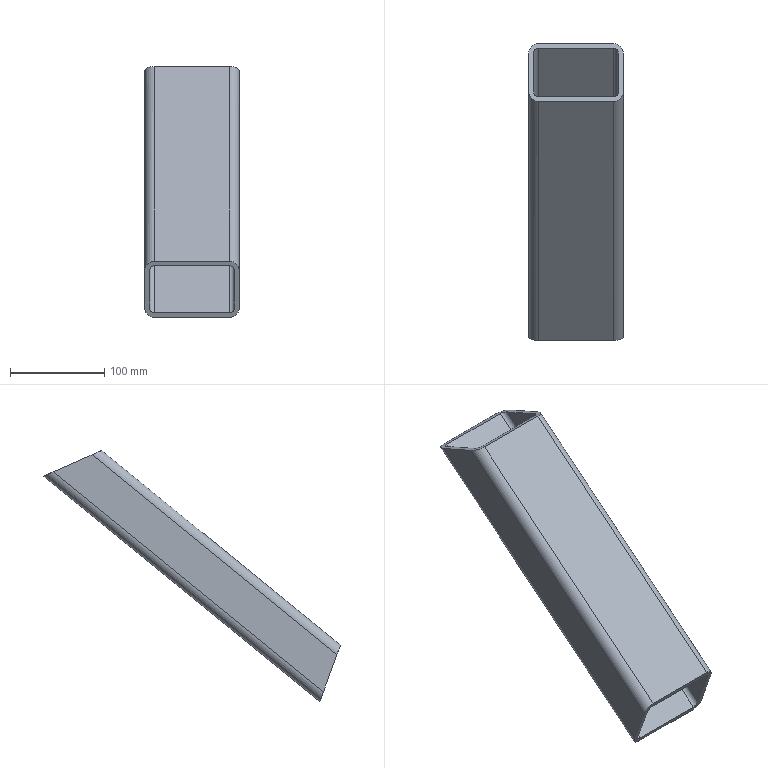Component | SolidWorks | Stap-2-8 | 1 solid | 18 faces | box 100 x 314.75 x 266.08 mm | volume 505822 mm3 | plane 10 | cylinder 8 | commonest cylinder face diameters 20 x4 10 x4 | material Plain Carbon Steel
build123d program:
from build123d import *

# Parameters (mm, degrees)
BOSS_EXTRUDE1_DEPTH = 100
FILLET1_R           = 10
SHELL1_T            = -5


with BuildPart() as part:
    # Sketch1 → Boss-Extrude1 (new body)
    with BuildSketch(Plane.XY):
        Polygon((1451.281, 1386.004), (1382.24, 1757.72), (1328.836, 1716.683), (1388.477, 1395.574), align=None)
    extrude(amount=BOSS_EXTRUDE1_DEPTH)

    # Fillet1
    fillet1_edges = [part.edges().sort_by_distance(p)[0] for p in [
        (1358.657, 1556.128, 100),
        (1358.657, 1556.128, 0),
        (1416.76, 1571.862, 0),
        (1416.76, 1571.862, 100),
    ]]
    fillet(fillet1_edges, radius=FILLET1_R)

    # Shell1
    shell1_openings = [part.faces().sort_by_distance(p)[0] for p in [
        (1355.538, 1737.202, 50),
        (1419.879, 1390.789, 50),
    ]]
    offset(amount=SHELL1_T, openings=shell1_openings, kind=Kind.INTERSECTION)


solid = part.part

# Placed as in the assembly
solid = solid.moved(Location((-124, -2903.176, 779.332), (28.67, 90, 0)))
STEP:
#1=COLOUR_RGB('',0.7922,0.8196,0.9333);
#2=FILL_AREA_STYLE_COLOUR('',#1);
#3=FILL_AREA_STYLE('',(#2));
#4=SURFACE_STYLE_FILL_AREA(#3);
#5=SURFACE_SIDE_STYLE('',(#4));
#6=SURFACE_STYLE_USAGE(.BOTH.,#5);
#7=PRESENTATION_STYLE_ASSIGNMENT((#6));
#8=CARTESIAN_POINT('',(-4.685,-39.722,8.689));
#9=VERTEX_POINT('',#8);
#10=CARTESIAN_POINT('',(-4.685,-39.151,7.122));
#11=VERTEX_POINT('',#10);
#12=CARTESIAN_POINT('',(-4.685,-39.865,9.08));
#13=DIRECTION('',(0.,0.3421,-0.9397));
#14=VECTOR('',#13,39.37);
#15=LINE('',#12,#14);
#16=EDGE_CURVE('',#9,#11,#15,.T.);
#17=ORIENTED_EDGE('',*,*,#16,.F.);
#18=CARTESIAN_POINT('',(-4.488,-39.793,8.884));
#19=VERTEX_POINT('',#18);
#20=CARTESIAN_POINT('',(-4.488,-39.793,8.884));
#21=CARTESIAN_POINT('',(-4.604,-39.793,8.884));
#22=CARTESIAN_POINT('',(-4.685,-39.764,8.803));
#23=CARTESIAN_POINT('',(-4.685,-39.722,8.689));
#24=(BOUNDED_CURVE()B_SPLINE_CURVE(3,(#20,#21,#22,#23),.UNSPECIFIED.,.F.,.T.)B_SPLINE_CURVE_WITH_KNOTS((4,4),(3.142,4.712),.UNSPECIFIED.)CURVE()GEOMETRIC_REPRESENTATION_ITEM()RATIONAL_B_SPLINE_CURVE((1.,0.8047,0.8047,1.))REPRESENTATION_ITEM(''));
#25=EDGE_CURVE('',#19,#9,#24,.T.);
#26=ORIENTED_EDGE('',*,*,#25,.F.);
#27=CARTESIAN_POINT('',(-1.339,-39.793,8.884));
#28=VERTEX_POINT('',#27);
#29=CARTESIAN_POINT('',(-0.9449,-39.793,8.884));
#30=DIRECTION('',(-1.,0.,-0.));
#31=VECTOR('',#30,39.37);
#32=LINE('',#29,#31);
#33=EDGE_CURVE('',#28,#19,#32,.T.);
#34=ORIENTED_EDGE('',*,*,#33,.F.);
#35=CARTESIAN_POINT('',(-1.142,-39.722,8.689));
#36=VERTEX_POINT('',#35);
#37=CARTESIAN_POINT('',(-1.142,-39.722,8.689));
#38=CARTESIAN_POINT('',(-1.142,-39.764,8.803));
#39=CARTESIAN_POINT('',(-1.223,-39.793,8.884));
#40=CARTESIAN_POINT('',(-1.339,-39.793,8.884));
#41=(BOUNDED_CURVE()B_SPLINE_CURVE(3,(#37,#38,#39,#40),.UNSPECIFIED.,.F.,.F.)B_SPLINE_CURVE_WITH_KNOTS((4,4),(4.712,6.283),.UNSPECIFIED.)CURVE()GEOMETRIC_REPRESENTATION_ITEM()RATIONAL_B_SPLINE_CURVE((1.,0.8047,0.8047,1.))REPRESENTATION_ITEM(''));
#42=EDGE_CURVE('',#36,#28,#41,.T.);
#43=ORIENTED_EDGE('',*,*,#42,.F.);
#44=CARTESIAN_POINT('',(-1.142,-39.151,7.122));
#45=VERTEX_POINT('',#44);
#46=CARTESIAN_POINT('',(-1.142,-39.865,9.08));
#47=DIRECTION('',(0.,0.3421,-0.9397));
#48=VECTOR('',#47,39.37);
#49=LINE('',#46,#48);
#50=EDGE_CURVE('',#36,#45,#49,.T.);
#51=ORIENTED_EDGE('',*,*,#50,.T.);
#52=CARTESIAN_POINT('',(-1.339,-39.08,6.926));
#53=VERTEX_POINT('',#52);
#54=CARTESIAN_POINT('',(-1.339,-39.08,6.926));
#55=CARTESIAN_POINT('',(-1.223,-39.08,6.926));
#56=CARTESIAN_POINT('',(-1.142,-39.11,7.007));
#57=CARTESIAN_POINT('',(-1.142,-39.151,7.122));
#58=(BOUNDED_CURVE()B_SPLINE_CURVE(3,(#54,#55,#56,#57),.UNSPECIFIED.,.F.,.F.)B_SPLINE_CURVE_WITH_KNOTS((4,4),(0.,1.571),.UNSPECIFIED.)CURVE()GEOMETRIC_REPRESENTATION_ITEM()RATIONAL_B_SPLINE_CURVE((1.,0.8047,0.8047,1.))REPRESENTATION_ITEM(''));
#59=EDGE_CURVE('',#53,#45,#58,.T.);
#60=ORIENTED_EDGE('',*,*,#59,.F.);
#61=CARTESIAN_POINT('',(-4.488,-39.08,6.926));
#62=VERTEX_POINT('',#61);
#63=CARTESIAN_POINT('',(-0.9449,-39.08,6.926));
#64=DIRECTION('',(-1.,0.,-0.));
#65=VECTOR('',#64,39.37);
#66=LINE('',#63,#65);
#67=EDGE_CURVE('',#53,#62,#66,.T.);
#68=ORIENTED_EDGE('',*,*,#67,.T.);
#69=CARTESIAN_POINT('',(-4.685,-39.151,7.122));
#70=CARTESIAN_POINT('',(-4.685,-39.11,7.007));
#71=CARTESIAN_POINT('',(-4.604,-39.08,6.926));
#72=CARTESIAN_POINT('',(-4.488,-39.08,6.926));
#73=(BOUNDED_CURVE()B_SPLINE_CURVE(3,(#69,#70,#71,#72),.UNSPECIFIED.,.F.,.T.)B_SPLINE_CURVE_WITH_KNOTS((4,4),(1.571,3.142),.UNSPECIFIED.)CURVE()GEOMETRIC_REPRESENTATION_ITEM()RATIONAL_B_SPLINE_CURVE((1.,0.8047,0.8047,1.))REPRESENTATION_ITEM(''));
#74=EDGE_CURVE('',#11,#62,#73,.T.);
#75=ORIENTED_EDGE('',*,*,#74,.F.);
#76=EDGE_LOOP('',(#17,#26,#34,#43,#51,#60,#68,#75));
#77=FACE_BOUND('',#76,.T.);
#78=CARTESIAN_POINT('',(-4.882,-39.722,8.689));
#79=VERTEX_POINT('',#78);
#80=CARTESIAN_POINT('',(-4.882,-39.151,7.122));
#81=VERTEX_POINT('',#80);
#82=CARTESIAN_POINT('',(-4.882,-39.865,9.08));
#83=DIRECTION('',(0.,0.3421,-0.9397));
#84=VECTOR('',#83,39.37);
#85=LINE('',#82,#84);
#86=EDGE_CURVE('',#79,#81,#85,.T.);
#87=ORIENTED_EDGE('',*,*,#86,.T.);
#88=CARTESIAN_POINT('',(-4.488,-39.009,6.73));
#89=VERTEX_POINT('',#88);
#90=CARTESIAN_POINT('',(-4.882,-39.151,7.122));
#91=CARTESIAN_POINT('',(-4.882,-39.068,6.892));
#92=CARTESIAN_POINT('',(-4.719,-39.009,6.73));
#93=CARTESIAN_POINT('',(-4.488,-39.009,6.73));
#94=(BOUNDED_CURVE()B_SPLINE_CURVE(3,(#90,#91,#92,#93),.UNSPECIFIED.,.F.,.T.)B_SPLINE_CURVE_WITH_KNOTS((4,4),(1.571,3.142),.UNSPECIFIED.)CURVE()GEOMETRIC_REPRESENTATION_ITEM()RATIONAL_B_SPLINE_CURVE((1.,0.8047,0.8047,1.))REPRESENTATION_ITEM(''));
#95=EDGE_CURVE('',#81,#89,#94,.T.);
#96=ORIENTED_EDGE('',*,*,#95,.T.);
#97=CARTESIAN_POINT('',(-1.339,-39.009,6.73));
#98=VERTEX_POINT('',#97);
#99=CARTESIAN_POINT('',(-0.9449,-39.009,6.73));
#100=DIRECTION('',(-1.,0.,-0.));
#101=VECTOR('',#100,39.37);
#102=LINE('',#99,#101);
#103=EDGE_CURVE('',#98,#89,#102,.T.);
#104=ORIENTED_EDGE('',*,*,#103,.F.);
#105=CARTESIAN_POINT('',(-0.9449,-39.151,7.122));
#106=VERTEX_POINT('',#105);
#107=CARTESIAN_POINT('',(-1.339,-39.009,6.73));
#108=CARTESIAN_POINT('',(-1.108,-39.009,6.73));
#109=CARTESIAN_POINT('',(-0.9449,-39.068,6.892));
#110=CARTESIAN_POINT('',(-0.9449,-39.151,7.122));
#111=(BOUNDED_CURVE()B_SPLINE_CURVE(3,(#107,#108,#109,#110),.UNSPECIFIED.,.F.,.F.)B_SPLINE_CURVE_WITH_KNOTS((4,4),(0.,1.571),.UNSPECIFIED.)CURVE()GEOMETRIC_REPRESENTATION_ITEM()RATIONAL_B_SPLINE_CURVE((1.,0.8047,0.8047,1.))REPRESENTATION_ITEM(''));
#112=EDGE_CURVE('',#98,#106,#111,.T.);
#113=ORIENTED_EDGE('',*,*,#112,.T.);
#114=CARTESIAN_POINT('',(-0.9449,-39.722,8.689));
#115=VERTEX_POINT('',#114);
#116=CARTESIAN_POINT('',(-0.9449,-39.865,9.08));
#117=DIRECTION('',(0.,0.3421,-0.9397));
#118=VECTOR('',#117,39.37);
#119=LINE('',#116,#118);
#120=EDGE_CURVE('',#115,#106,#119,.T.);
#121=ORIENTED_EDGE('',*,*,#120,.F.);
#122=CARTESIAN_POINT('',(-1.339,-39.865,9.08));
#123=VERTEX_POINT('',#122);
#124=CARTESIAN_POINT('',(-0.9449,-39.722,8.689));
#125=CARTESIAN_POINT('',(-0.9449,-39.805,8.918));
#126=CARTESIAN_POINT('',(-1.108,-39.865,9.08));
#127=CARTESIAN_POINT('',(-1.339,-39.865,9.08));
#128=(BOUNDED_CURVE()B_SPLINE_CURVE(3,(#124,#125,#126,#127),.UNSPECIFIED.,.F.,.T.)B_SPLINE_CURVE_WITH_KNOTS((4,4),(4.712,6.283),.UNSPECIFIED.)CURVE()GEOMETRIC_REPRESENTATION_ITEM()RATIONAL_B_SPLINE_CURVE((1.,0.8047,0.8047,1.))REPRESENTATION_ITEM(''));
#129=EDGE_CURVE('',#115,#123,#128,.T.);
#130=ORIENTED_EDGE('',*,*,#129,.T.);
#131=CARTESIAN_POINT('',(-4.488,-39.865,9.08));
#132=VERTEX_POINT('',#131);
#133=CARTESIAN_POINT('',(-0.9449,-39.865,9.08));
#134=DIRECTION('',(-1.,0.,-0.));
#135=VECTOR('',#134,39.37);
#136=LINE('',#133,#135);
#137=EDGE_CURVE('',#123,#132,#136,.T.);
#138=ORIENTED_EDGE('',*,*,#137,.T.);
#139=CARTESIAN_POINT('',(-4.488,-39.865,9.08));
#140=CARTESIAN_POINT('',(-4.719,-39.865,9.08));
#141=CARTESIAN_POINT('',(-4.882,-39.805,8.918));
#142=CARTESIAN_POINT('',(-4.882,-39.722,8.689));
#143=(BOUNDED_CURVE()B_SPLINE_CURVE(3,(#139,#140,#141,#142),.UNSPECIFIED.,.F.,.F.)B_SPLINE_CURVE_WITH_KNOTS((4,4),(3.142,4.712),.UNSPECIFIED.)CURVE()GEOMETRIC_REPRESENTATION_ITEM()RATIONAL_B_SPLINE_CURVE((1.,0.8047,0.8047,1.))REPRESENTATION_ITEM(''));
#144=EDGE_CURVE('',#132,#79,#143,.T.);
#145=ORIENTED_EDGE('',*,*,#144,.T.);
#146=EDGE_LOOP('',(#87,#96,#104,#113,#121,#130,#138,#145));
#147=FACE_OUTER_BOUND('',#146,.T.);
#148=CARTESIAN_POINT('',(-0.9449,-39.865,9.08));
#149=DIRECTION('',(-0.,0.9397,0.3421));
#150=DIRECTION('',(-0.,-0.3421,0.9397));
#151=AXIS2_PLACEMENT_3D('',#148,#149,#150);
#152=PLANE('',#151);
#153=ADVANCED_FACE('',(#77,#147),#152,.F.);
#154=ORIENTED_EDGE('',*,*,#103,.T.);
#155=CARTESIAN_POINT('',(-4.488,-27.473,16.136));
#156=VERTEX_POINT('',#155);
#157=CARTESIAN_POINT('',(-4.488,-39.009,6.73));
#158=DIRECTION('',(-0.,0.775,0.6319));
#159=VECTOR('',#158,39.37);
#160=LINE('',#157,#159);
#161=EDGE_CURVE('',#89,#156,#160,.T.);
#162=ORIENTED_EDGE('',*,*,#161,.T.);
#163=CARTESIAN_POINT('',(-1.339,-27.473,16.136));
#164=VERTEX_POINT('',#163);
#165=CARTESIAN_POINT('',(-0.9449,-27.473,16.136));
#166=DIRECTION('',(-1.,0.,-0.));
#167=VECTOR('',#166,39.37);
#168=LINE('',#165,#167);
#169=EDGE_CURVE('',#164,#156,#168,.T.);
#170=ORIENTED_EDGE('',*,*,#169,.F.);
#171=CARTESIAN_POINT('',(-1.339,-39.009,6.73));
#172=DIRECTION('',(0.,-0.775,-0.6319));
#173=VECTOR('',#172,39.37);
#174=LINE('',#171,#173);
#175=EDGE_CURVE('',#164,#98,#174,.T.);
#176=ORIENTED_EDGE('',*,*,#175,.T.);
#177=EDGE_LOOP('',(#154,#162,#170,#176));
#178=FACE_OUTER_BOUND('',#177,.T.);
#179=CARTESIAN_POINT('',(-0.9449,-39.009,6.73));
#180=DIRECTION('',(-0.,-0.6319,0.775));
#181=DIRECTION('',(0.,-0.775,-0.6319));
#182=AXIS2_PLACEMENT_3D('',#179,#180,#181);
#183=PLANE('',#182);
#184=ADVANCED_FACE('',(#178),#183,.F.);
#185=CARTESIAN_POINT('',(-1.339,-27.675,16.225));
#186=VERTEX_POINT('',#185);
#187=CARTESIAN_POINT('',(-4.488,-27.675,16.225));
#188=VERTEX_POINT('',#187);
#189=CARTESIAN_POINT('',(-0.9449,-27.675,16.225));
#190=DIRECTION('',(-1.,0.,-0.));
#191=VECTOR('',#190,39.37);
#192=LINE('',#189,#191);
#193=EDGE_CURVE('',#186,#188,#192,.T.);
#194=ORIENTED_EDGE('',*,*,#193,.F.);
#195=CARTESIAN_POINT('',(-1.142,-27.877,16.314));
#196=VERTEX_POINT('',#195);
#197=CARTESIAN_POINT('',(-1.142,-27.877,16.314));
#198=CARTESIAN_POINT('',(-1.142,-27.759,16.262));
#199=CARTESIAN_POINT('',(-1.223,-27.675,16.225));
#200=CARTESIAN_POINT('',(-1.339,-27.675,16.225));
#201=(BOUNDED_CURVE()B_SPLINE_CURVE(3,(#197,#198,#199,#200),.UNSPECIFIED.,.F.,.T.)B_SPLINE_CURVE_WITH_KNOTS((4,4),(1.571,3.142),.UNSPECIFIED.)CURVE()GEOMETRIC_REPRESENTATION_ITEM()RATIONAL_B_SPLINE_CURVE((1.,0.8047,0.8047,1.))REPRESENTATION_ITEM(''));
#202=EDGE_CURVE('',#196,#186,#201,.T.);
#203=ORIENTED_EDGE('',*,*,#202,.F.);
#204=CARTESIAN_POINT('',(-1.142,-29.495,17.027));
#205=VERTEX_POINT('',#204);
#206=CARTESIAN_POINT('',(-1.142,-27.473,16.136));
#207=DIRECTION('',(-0.,-0.915,0.4034));
#208=VECTOR('',#207,39.37);
#209=LINE('',#206,#208);
#210=EDGE_CURVE('',#196,#205,#209,.T.);
#211=ORIENTED_EDGE('',*,*,#210,.T.);
#212=CARTESIAN_POINT('',(-1.339,-29.697,17.117));
#213=VERTEX_POINT('',#212);
#214=CARTESIAN_POINT('',(-1.339,-29.697,17.117));
#215=CARTESIAN_POINT('',(-1.223,-29.697,17.117));
#216=CARTESIAN_POINT('',(-1.142,-29.613,17.08));
#217=CARTESIAN_POINT('',(-1.142,-29.495,17.027));
#218=(BOUNDED_CURVE()B_SPLINE_CURVE(3,(#214,#215,#216,#217),.UNSPECIFIED.,.F.,.T.)B_SPLINE_CURVE_WITH_KNOTS((4,4),(3.142,4.712),.UNSPECIFIED.)CURVE()GEOMETRIC_REPRESENTATION_ITEM()RATIONAL_B_SPLINE_CURVE((1.,0.8047,0.8047,1.))REPRESENTATION_ITEM(''));
#219=EDGE_CURVE('',#213,#205,#218,.T.);
#220=ORIENTED_EDGE('',*,*,#219,.F.);
#221=CARTESIAN_POINT('',(-4.488,-29.697,17.117));
#222=VERTEX_POINT('',#221);
#223=CARTESIAN_POINT('',(-0.9449,-29.697,17.117));
#224=DIRECTION('',(-1.,0.,-0.));
#225=VECTOR('',#224,39.37);
#226=LINE('',#223,#225);
#227=EDGE_CURVE('',#213,#222,#226,.T.);
#228=ORIENTED_EDGE('',*,*,#227,.T.);
#229=CARTESIAN_POINT('',(-4.685,-29.495,17.027));
#230=VERTEX_POINT('',#229);
#231=CARTESIAN_POINT('',(-4.685,-29.495,17.027));
#232=CARTESIAN_POINT('',(-4.685,-29.613,17.08));
#233=CARTESIAN_POINT('',(-4.604,-29.697,17.117));
#234=CARTESIAN_POINT('',(-4.488,-29.697,17.117));
#235=(BOUNDED_CURVE()B_SPLINE_CURVE(3,(#231,#232,#233,#234),.UNSPECIFIED.,.F.,.T.)B_SPLINE_CURVE_WITH_KNOTS((4,4),(4.712,6.283),.UNSPECIFIED.)CURVE()GEOMETRIC_REPRESENTATION_ITEM()RATIONAL_B_SPLINE_CURVE((1.,0.8047,0.8047,1.))REPRESENTATION_ITEM(''));
#236=EDGE_CURVE('',#230,#222,#235,.T.);
#237=ORIENTED_EDGE('',*,*,#236,.F.);
#238=CARTESIAN_POINT('',(-4.685,-27.877,16.314));
#239=VERTEX_POINT('',#238);
#240=CARTESIAN_POINT('',(-4.685,-27.473,16.136));
#241=DIRECTION('',(-0.,-0.915,0.4034));
#242=VECTOR('',#241,39.37);
#243=LINE('',#240,#242);
#244=EDGE_CURVE('',#239,#230,#243,.T.);
#245=ORIENTED_EDGE('',*,*,#244,.F.);
#246=CARTESIAN_POINT('',(-4.488,-27.675,16.225));
#247=CARTESIAN_POINT('',(-4.604,-27.675,16.225));
#248=CARTESIAN_POINT('',(-4.685,-27.759,16.262));
#249=CARTESIAN_POINT('',(-4.685,-27.877,16.314));
#250=(BOUNDED_CURVE()B_SPLINE_CURVE(3,(#246,#247,#248,#249),.UNSPECIFIED.,.F.,.T.)B_SPLINE_CURVE_WITH_KNOTS((4,4),(0.,1.571),.UNSPECIFIED.)CURVE()GEOMETRIC_REPRESENTATION_ITEM()RATIONAL_B_SPLINE_CURVE((1.,0.8047,0.8047,1.))REPRESENTATION_ITEM(''));
#251=EDGE_CURVE('',#188,#239,#250,.T.);
#252=ORIENTED_EDGE('',*,*,#251,.F.);
#253=EDGE_LOOP('',(#194,#203,#211,#220,#228,#237,#245,#252));
#254=FACE_BOUND('',#253,.T.);
#255=ORIENTED_EDGE('',*,*,#169,.T.);
#256=CARTESIAN_POINT('',(-4.882,-27.877,16.314));
#257=VERTEX_POINT('',#256);
#258=CARTESIAN_POINT('',(-4.488,-27.473,16.136));
#259=CARTESIAN_POINT('',(-4.719,-27.473,16.136));
#260=CARTESIAN_POINT('',(-4.882,-27.64,16.21));
#261=CARTESIAN_POINT('',(-4.882,-27.877,16.314));
#262=(BOUNDED_CURVE()B_SPLINE_CURVE(3,(#258,#259,#260,#261),.UNSPECIFIED.,.F.,.F.)B_SPLINE_CURVE_WITH_KNOTS((4,4),(0.,1.571),.UNSPECIFIED.)CURVE()GEOMETRIC_REPRESENTATION_ITEM()RATIONAL_B_SPLINE_CURVE((1.,0.8047,0.8047,1.))REPRESENTATION_ITEM(''));
#263=EDGE_CURVE('',#156,#257,#262,.T.);
#264=ORIENTED_EDGE('',*,*,#263,.T.);
#265=CARTESIAN_POINT('',(-4.882,-29.495,17.027));
#266=VERTEX_POINT('',#265);
#267=CARTESIAN_POINT('',(-4.882,-27.473,16.136));
#268=DIRECTION('',(-0.,-0.915,0.4034));
#269=VECTOR('',#268,39.37);
#270=LINE('',#267,#269);
#271=EDGE_CURVE('',#257,#266,#270,.T.);
#272=ORIENTED_EDGE('',*,*,#271,.T.);
#273=CARTESIAN_POINT('',(-4.488,-29.899,17.206));
#274=VERTEX_POINT('',#273);
#275=CARTESIAN_POINT('',(-4.882,-29.495,17.027));
#276=CARTESIAN_POINT('',(-4.882,-29.731,17.132));
#277=CARTESIAN_POINT('',(-4.719,-29.899,17.206));
#278=CARTESIAN_POINT('',(-4.488,-29.899,17.206));
#279=(BOUNDED_CURVE()B_SPLINE_CURVE(3,(#275,#276,#277,#278),.UNSPECIFIED.,.F.,.T.)B_SPLINE_CURVE_WITH_KNOTS((4,4),(4.712,6.283),.UNSPECIFIED.)CURVE()GEOMETRIC_REPRESENTATION_ITEM()RATIONAL_B_SPLINE_CURVE((1.,0.8047,0.8047,1.))REPRESENTATION_ITEM(''));
#280=EDGE_CURVE('',#266,#274,#279,.T.);
#281=ORIENTED_EDGE('',*,*,#280,.T.);
#282=CARTESIAN_POINT('',(-1.339,-29.899,17.206));
#283=VERTEX_POINT('',#282);
#284=CARTESIAN_POINT('',(-0.9449,-29.899,17.206));
#285=DIRECTION('',(-1.,0.,-0.));
#286=VECTOR('',#285,39.37);
#287=LINE('',#284,#286);
#288=EDGE_CURVE('',#283,#274,#287,.T.);
#289=ORIENTED_EDGE('',*,*,#288,.F.);
#290=CARTESIAN_POINT('',(-0.9449,-29.495,17.027));
#291=VERTEX_POINT('',#290);
#292=CARTESIAN_POINT('',(-1.339,-29.899,17.206));
#293=CARTESIAN_POINT('',(-1.108,-29.899,17.206));
#294=CARTESIAN_POINT('',(-0.9449,-29.731,17.132));
#295=CARTESIAN_POINT('',(-0.9449,-29.495,17.027));
#296=(BOUNDED_CURVE()B_SPLINE_CURVE(3,(#292,#293,#294,#295),.UNSPECIFIED.,.F.,.T.)B_SPLINE_CURVE_WITH_KNOTS((4,4),(3.142,4.712),.UNSPECIFIED.)CURVE()GEOMETRIC_REPRESENTATION_ITEM()RATIONAL_B_SPLINE_CURVE((1.,0.8047,0.8047,1.))REPRESENTATION_ITEM(''));
#297=EDGE_CURVE('',#283,#291,#296,.T.);
#298=ORIENTED_EDGE('',*,*,#297,.T.);
#299=CARTESIAN_POINT('',(-0.9449,-27.877,16.314));
#300=VERTEX_POINT('',#299);
#301=CARTESIAN_POINT('',(-0.9449,-27.473,16.136));
#302=DIRECTION('',(-0.,-0.915,0.4034));
#303=VECTOR('',#302,39.37);
#304=LINE('',#301,#303);
#305=EDGE_CURVE('',#300,#291,#304,.T.);
#306=ORIENTED_EDGE('',*,*,#305,.F.);
#307=CARTESIAN_POINT('',(-0.9449,-27.877,16.314));
#308=CARTESIAN_POINT('',(-0.9449,-27.64,16.21));
#309=CARTESIAN_POINT('',(-1.108,-27.473,16.136));
#310=CARTESIAN_POINT('',(-1.339,-27.473,16.136));
#311=(BOUNDED_CURVE()B_SPLINE_CURVE(3,(#307,#308,#309,#310),.UNSPECIFIED.,.F.,.T.)B_SPLINE_CURVE_WITH_KNOTS((4,4),(1.571,3.142),.UNSPECIFIED.)CURVE()GEOMETRIC_REPRESENTATION_ITEM()RATIONAL_B_SPLINE_CURVE((1.,0.8047,0.8047,1.))REPRESENTATION_ITEM(''));
#312=EDGE_CURVE('',#300,#164,#311,.T.);
#313=ORIENTED_EDGE('',*,*,#312,.T.);
#314=EDGE_LOOP('',(#255,#264,#272,#281,#289,#298,#306,#313));
#315=FACE_OUTER_BOUND('',#314,.T.);
#316=CARTESIAN_POINT('',(-0.9449,-27.473,16.136));
#317=DIRECTION('',(0.,-0.4034,-0.915));
#318=DIRECTION('',(0.,0.915,-0.4034));
#319=AXIS2_PLACEMENT_3D('',#316,#317,#318);
#320=PLANE('',#319);
#321=ADVANCED_FACE('',(#254,#315),#320,.F.);
#322=ORIENTED_EDGE('',*,*,#288,.T.);
#323=CARTESIAN_POINT('',(-4.488,-29.899,17.206));
#324=DIRECTION('',(0.,-0.775,-0.6319));
#325=VECTOR('',#324,39.37);
#326=LINE('',#323,#325);
#327=EDGE_CURVE('',#274,#132,#326,.T.);
#328=ORIENTED_EDGE('',*,*,#327,.T.);
#329=ORIENTED_EDGE('',*,*,#137,.F.);
#330=CARTESIAN_POINT('',(-1.339,-29.899,17.206));
#331=DIRECTION('',(-0.,0.775,0.6319));
#332=VECTOR('',#331,39.37);
#333=LINE('',#330,#332);
#334=EDGE_CURVE('',#123,#283,#333,.T.);
#335=ORIENTED_EDGE('',*,*,#334,.T.);
#336=EDGE_LOOP('',(#322,#328,#329,#335));
#337=FACE_OUTER_BOUND('',#336,.T.);
#338=CARTESIAN_POINT('',(-0.9449,-29.899,17.206));
#339=DIRECTION('',(0.,0.6319,-0.775));
#340=DIRECTION('',(-0.,0.775,0.6319));
#341=AXIS2_PLACEMENT_3D('',#338,#339,#340);
#342=PLANE('',#341);
#343=ADVANCED_FACE('',(#337),#342,.F.);
#344=ORIENTED_EDGE('',*,*,#120,.T.);
#345=CARTESIAN_POINT('',(-0.9449,-27.721,16.441));
#346=DIRECTION('',(-0.,0.775,0.6319));
#347=VECTOR('',#346,39.37);
#348=LINE('',#345,#347);
#349=EDGE_CURVE('',#106,#300,#348,.T.);
#350=ORIENTED_EDGE('',*,*,#349,.T.);
#351=ORIENTED_EDGE('',*,*,#305,.T.);
#352=CARTESIAN_POINT('',(-0.9449,-39.616,8.775));
#353=DIRECTION('',(0.,-0.775,-0.6319));
#354=VECTOR('',#353,39.37);
#355=LINE('',#352,#354);
#356=EDGE_CURVE('',#291,#115,#355,.T.);
#357=ORIENTED_EDGE('',*,*,#356,.T.);
#358=EDGE_LOOP('',(#344,#350,#351,#357));
#359=FACE_OUTER_BOUND('',#358,.T.);
#360=CARTESIAN_POINT('',(-0.9449,-114.298,30.682));
#361=DIRECTION('',(1.,-0.,0.));
#362=DIRECTION('',(0.,0.4798,-0.8774));
#363=AXIS2_PLACEMENT_3D('',#360,#361,#362);
#364=PLANE('',#363);
#365=ADVANCED_FACE('',(#359),#364,.T.);
#366=ORIENTED_EDGE('',*,*,#271,.F.);
#367=CARTESIAN_POINT('',(-4.882,-72.751,-20.274));
#368=DIRECTION('',(0.,-0.775,-0.6319));
#369=VECTOR('',#368,39.37);
#370=LINE('',#367,#369);
#371=EDGE_CURVE('',#257,#81,#370,.T.);
#372=ORIENTED_EDGE('',*,*,#371,.T.);
#373=ORIENTED_EDGE('',*,*,#86,.F.);
#374=CARTESIAN_POINT('',(-4.882,-73.746,-19.053));
#375=DIRECTION('',(-0.,0.775,0.6319));
#376=VECTOR('',#375,39.37);
#377=LINE('',#374,#376);
#378=EDGE_CURVE('',#79,#266,#377,.T.);
#379=ORIENTED_EDGE('',*,*,#378,.T.);
#380=EDGE_LOOP('',(#366,#372,#373,#379));
#381=FACE_OUTER_BOUND('',#380,.T.);
#382=CARTESIAN_POINT('',(-4.882,-114.298,30.682));
#383=DIRECTION('',(1.,-0.,0.));
#384=DIRECTION('',(0.,0.4798,-0.8774));
#385=AXIS2_PLACEMENT_3D('',#382,#383,#384);
#386=PLANE('',#385);
#387=ADVANCED_FACE('',(#381),#386,.F.);
#388=ORIENTED_EDGE('',*,*,#95,.F.);
#389=ORIENTED_EDGE('',*,*,#371,.F.);
#390=ORIENTED_EDGE('',*,*,#263,.F.);
#391=ORIENTED_EDGE('',*,*,#161,.F.);
#392=EDGE_LOOP('',(#388,#389,#390,#391));
#393=FACE_OUTER_BOUND('',#392,.T.);
#394=CARTESIAN_POINT('',(-4.488,-39.258,7.035));
#395=DIRECTION('',(-0.,0.775,0.6319));
#396=DIRECTION('',(0.,-0.6319,0.775));
#397=AXIS2_PLACEMENT_3D('',#394,#395,#396);
#398=CYLINDRICAL_SURFACE('',#397,0.3937);
#399=ADVANCED_FACE('',(#393),#398,.T.);
#400=ORIENTED_EDGE('',*,*,#280,.F.);
#401=ORIENTED_EDGE('',*,*,#378,.F.);
#402=ORIENTED_EDGE('',*,*,#144,.F.);
#403=ORIENTED_EDGE('',*,*,#327,.F.);
#404=EDGE_LOOP('',(#400,#401,#402,#403));
#405=FACE_OUTER_BOUND('',#404,.T.);
#406=CARTESIAN_POINT('',(-4.488,-29.65,16.901));
#407=DIRECTION('',(0.,-0.775,-0.6319));
#408=DIRECTION('',(0.,0.6319,-0.775));
#409=AXIS2_PLACEMENT_3D('',#406,#407,#408);
#410=CYLINDRICAL_SURFACE('',#409,0.3937);
#411=ADVANCED_FACE('',(#405),#410,.T.);
#412=ORIENTED_EDGE('',*,*,#112,.F.);
#413=ORIENTED_EDGE('',*,*,#175,.F.);
#414=ORIENTED_EDGE('',*,*,#312,.F.);
#415=ORIENTED_EDGE('',*,*,#349,.F.);
#416=EDGE_LOOP('',(#412,#413,#414,#415));
#417=FACE_OUTER_BOUND('',#416,.T.);
#418=CARTESIAN_POINT('',(-1.339,-72.751,-20.274));
#419=DIRECTION('',(0.,-0.775,-0.6319));
#420=DIRECTION('',(0.,0.6319,-0.775));
#421=AXIS2_PLACEMENT_3D('',#418,#419,#420);
#422=CYLINDRICAL_SURFACE('',#421,0.3937);
#423=ADVANCED_FACE('',(#417),#422,.T.);
#424=ORIENTED_EDGE('',*,*,#297,.F.);
#425=ORIENTED_EDGE('',*,*,#334,.F.);
#426=ORIENTED_EDGE('',*,*,#129,.F.);
#427=ORIENTED_EDGE('',*,*,#356,.F.);
#428=EDGE_LOOP('',(#424,#425,#426,#427));
#429=FACE_OUTER_BOUND('',#428,.T.);
#430=CARTESIAN_POINT('',(-1.339,-73.746,-19.053));
#431=DIRECTION('',(-0.,0.775,0.6319));
#432=DIRECTION('',(0.,-0.6319,0.775));
#433=AXIS2_PLACEMENT_3D('',#430,#431,#432);
#434=CYLINDRICAL_SURFACE('',#433,0.3937);
#435=ADVANCED_FACE('',(#429),#434,.T.);
#436=ORIENTED_EDGE('',*,*,#67,.F.);
#437=CARTESIAN_POINT('',(-1.339,-39.133,6.883));
#438=DIRECTION('',(0.,-0.775,-0.6319));
#439=VECTOR('',#438,39.37);
#440=LINE('',#437,#439);
#441=EDGE_CURVE('',#186,#53,#440,.T.);
#442=ORIENTED_EDGE('',*,*,#441,.F.);
#443=ORIENTED_EDGE('',*,*,#193,.T.);
#444=CARTESIAN_POINT('',(-4.488,-39.133,6.883));
#445=DIRECTION('',(-0.,0.775,0.6319));
#446=VECTOR('',#445,39.37);
#447=LINE('',#444,#446);
#448=EDGE_CURVE('',#62,#188,#447,.T.);
#449=ORIENTED_EDGE('',*,*,#448,.F.);
#450=EDGE_LOOP('',(#436,#442,#443,#449));
#451=FACE_OUTER_BOUND('',#450,.T.);
#452=CARTESIAN_POINT('',(-0.9449,-39.133,6.883));
#453=DIRECTION('',(-0.,-0.6319,0.775));
#454=DIRECTION('',(0.,-0.775,-0.6319));
#455=AXIS2_PLACEMENT_3D('',#452,#453,#454);
#456=PLANE('',#455);
#457=ADVANCED_FACE('',(#451),#456,.T.);
#458=ORIENTED_EDGE('',*,*,#227,.F.);
#459=CARTESIAN_POINT('',(-1.339,-29.775,17.053));
#460=DIRECTION('',(-0.,0.775,0.6319));
#461=VECTOR('',#460,39.37);
#462=LINE('',#459,#461);
#463=EDGE_CURVE('',#28,#213,#462,.T.);
#464=ORIENTED_EDGE('',*,*,#463,.F.);
#465=ORIENTED_EDGE('',*,*,#33,.T.);
#466=CARTESIAN_POINT('',(-4.488,-29.775,17.053));
#467=DIRECTION('',(0.,-0.775,-0.6319));
#468=VECTOR('',#467,39.37);
#469=LINE('',#466,#468);
#470=EDGE_CURVE('',#222,#19,#469,.T.);
#471=ORIENTED_EDGE('',*,*,#470,.F.);
#472=EDGE_LOOP('',(#458,#464,#465,#471));
#473=FACE_OUTER_BOUND('',#472,.T.);
#474=CARTESIAN_POINT('',(-0.9449,-29.775,17.053));
#475=DIRECTION('',(0.,0.6319,-0.775));
#476=DIRECTION('',(-0.,0.775,0.6319));
#477=AXIS2_PLACEMENT_3D('',#474,#475,#476);
#478=PLANE('',#477);
#479=ADVANCED_FACE('',(#473),#478,.T.);
#480=ORIENTED_EDGE('',*,*,#50,.F.);
#481=CARTESIAN_POINT('',(-1.142,-73.746,-19.053));
#482=DIRECTION('',(0.,-0.775,-0.6319));
#483=VECTOR('',#482,39.37);
#484=LINE('',#481,#483);
#485=EDGE_CURVE('',#205,#36,#484,.T.);
#486=ORIENTED_EDGE('',*,*,#485,.F.);
#487=ORIENTED_EDGE('',*,*,#210,.F.);
#488=CARTESIAN_POINT('',(-1.142,-72.751,-20.274));
#489=DIRECTION('',(-0.,0.775,0.6319));
#490=VECTOR('',#489,39.37);
#491=LINE('',#488,#490);
#492=EDGE_CURVE('',#45,#196,#491,.T.);
#493=ORIENTED_EDGE('',*,*,#492,.F.);
#494=EDGE_LOOP('',(#480,#486,#487,#493));
#495=FACE_OUTER_BOUND('',#494,.T.);
#496=CARTESIAN_POINT('',(-1.142,-114.298,30.682));
#497=DIRECTION('',(1.,-0.,0.));
#498=DIRECTION('',(0.,0.4798,-0.8774));
#499=AXIS2_PLACEMENT_3D('',#496,#497,#498);
#500=PLANE('',#499);
#501=ADVANCED_FACE('',(#495),#500,.F.);
#502=ORIENTED_EDGE('',*,*,#244,.T.);
#503=CARTESIAN_POINT('',(-4.685,-29.65,16.901));
#504=DIRECTION('',(-0.,0.775,0.6319));
#505=VECTOR('',#504,39.37);
#506=LINE('',#503,#505);
#507=EDGE_CURVE('',#9,#230,#506,.T.);
#508=ORIENTED_EDGE('',*,*,#507,.F.);
#509=ORIENTED_EDGE('',*,*,#16,.T.);
#510=CARTESIAN_POINT('',(-4.685,-39.258,7.035));
#511=DIRECTION('',(0.,-0.775,-0.6319));
#512=VECTOR('',#511,39.37);
#513=LINE('',#510,#512);
#514=EDGE_CURVE('',#239,#11,#513,.T.);
#515=ORIENTED_EDGE('',*,*,#514,.F.);
#516=EDGE_LOOP('',(#502,#508,#509,#515));
#517=FACE_OUTER_BOUND('',#516,.T.);
#518=CARTESIAN_POINT('',(-4.685,-114.298,30.682));
#519=DIRECTION('',(1.,-0.,0.));
#520=DIRECTION('',(0.,0.4798,-0.8774));
#521=AXIS2_PLACEMENT_3D('',#518,#519,#520);
#522=PLANE('',#521);
#523=ADVANCED_FACE('',(#517),#522,.T.);
#524=ORIENTED_EDGE('',*,*,#74,.T.);
#525=ORIENTED_EDGE('',*,*,#448,.T.);
#526=ORIENTED_EDGE('',*,*,#251,.T.);
#527=ORIENTED_EDGE('',*,*,#514,.T.);
#528=EDGE_LOOP('',(#524,#525,#526,#527));
#529=FACE_OUTER_BOUND('',#528,.T.);
#530=CARTESIAN_POINT('',(-4.488,-39.258,7.035));
#531=DIRECTION('',(-0.,0.775,0.6319));
#532=DIRECTION('',(0.,-0.6319,0.775));
#533=AXIS2_PLACEMENT_3D('',#530,#531,#532);
#534=CYLINDRICAL_SURFACE('',#533,0.1969);
#535=ADVANCED_FACE('',(#529),#534,.F.);
#536=ORIENTED_EDGE('',*,*,#236,.T.);
#537=ORIENTED_EDGE('',*,*,#470,.T.);
#538=ORIENTED_EDGE('',*,*,#25,.T.);
#539=ORIENTED_EDGE('',*,*,#507,.T.);
#540=EDGE_LOOP('',(#536,#537,#538,#539));
#541=FACE_OUTER_BOUND('',#540,.T.);
#542=CARTESIAN_POINT('',(-4.488,-29.65,16.901));
#543=DIRECTION('',(0.,-0.775,-0.6319));
#544=DIRECTION('',(0.,0.6319,-0.775));
#545=AXIS2_PLACEMENT_3D('',#542,#543,#544);
#546=CYLINDRICAL_SURFACE('',#545,0.1969);
#547=ADVANCED_FACE('',(#541),#546,.F.);
#548=ORIENTED_EDGE('',*,*,#59,.T.);
#549=ORIENTED_EDGE('',*,*,#492,.T.);
#550=ORIENTED_EDGE('',*,*,#202,.T.);
#551=ORIENTED_EDGE('',*,*,#441,.T.);
#552=EDGE_LOOP('',(#548,#549,#550,#551));
#553=FACE_OUTER_BOUND('',#552,.T.);
#554=CARTESIAN_POINT('',(-1.339,-72.751,-20.274));
#555=DIRECTION('',(0.,-0.775,-0.6319));
#556=DIRECTION('',(0.,0.6319,-0.775));
#557=AXIS2_PLACEMENT_3D('',#554,#555,#556);
#558=CYLINDRICAL_SURFACE('',#557,0.1969);
#559=ADVANCED_FACE('',(#553),#558,.F.);
#560=ORIENTED_EDGE('',*,*,#219,.T.);
#561=ORIENTED_EDGE('',*,*,#485,.T.);
#562=ORIENTED_EDGE('',*,*,#42,.T.);
#563=ORIENTED_EDGE('',*,*,#463,.T.);
#564=EDGE_LOOP('',(#560,#561,#562,#563));
#565=FACE_OUTER_BOUND('',#564,.T.);
#566=CARTESIAN_POINT('',(-1.339,-73.746,-19.053));
#567=DIRECTION('',(-0.,0.775,0.6319));
#568=DIRECTION('',(0.,-0.6319,0.775));
#569=AXIS2_PLACEMENT_3D('',#566,#567,#568);
#570=CYLINDRICAL_SURFACE('',#569,0.1969);
#571=ADVANCED_FACE('',(#565),#570,.F.);
#572=CLOSED_SHELL('',(#153,#184,#321,#343,#365,#387,#399,#411,#423,#435,#457,#479,#501,#523,#535,#547,#559,#571));
#573=MANIFOLD_SOLID_BREP('',#572);
#574=STYLED_ITEM('',(#7),#573);
#575=(LENGTH_UNIT()NAMED_UNIT(*)SI_UNIT($,.METRE.));
#576=LENGTH_MEASURE_WITH_UNIT(LENGTH_MEASURE(0.0254),#575);
#577=DIMENSIONAL_EXPONENTS(1.,0.,0.,0.,0.,0.,0.);
#578=(CONVERSION_BASED_UNIT('',#576)LENGTH_UNIT()NAMED_UNIT(#577));
#579=UNCERTAINTY_MEASURE_WITH_UNIT(LENGTH_MEASURE(0.00001),#578,'','');
#580=(NAMED_UNIT(*)PLANE_ANGLE_UNIT()SI_UNIT($,.RADIAN.));
#581=(NAMED_UNIT(*)SI_UNIT($,.STERADIAN.)SOLID_ANGLE_UNIT());
#582=(GEOMETRIC_REPRESENTATION_CONTEXT(3)GLOBAL_UNCERTAINTY_ASSIGNED_CONTEXT((#579))GLOBAL_UNIT_ASSIGNED_CONTEXT((#578,#580,#581))REPRESENTATION_CONTEXT('',''));
#583=MECHANICAL_DESIGN_GEOMETRIC_PRESENTATION_REPRESENTATION('',(#574),#582);
#584=PRESENTATION_LAYER_ASSIGNMENT('','',(#574));
#585=CARTESIAN_POINT('',(0.,0.,0.));
#586=DIRECTION('',(0.,0.,1.));
#587=DIRECTION('',(1.,0.,0.));
#588=AXIS2_PLACEMENT_3D('',#585,#586,#587);
#589=(LENGTH_UNIT()NAMED_UNIT(*)SI_UNIT($,.METRE.));
#590=LENGTH_MEASURE_WITH_UNIT(LENGTH_MEASURE(0.0254),#589);
#591=DIMENSIONAL_EXPONENTS(1.,0.,0.,0.,0.,0.,0.);
#592=(CONVERSION_BASED_UNIT('',#590)LENGTH_UNIT()NAMED_UNIT(#591));
#593=UNCERTAINTY_MEASURE_WITH_UNIT(LENGTH_MEASURE(0.00001),#592,'','');
#594=(NAMED_UNIT(*)PLANE_ANGLE_UNIT()SI_UNIT($,.RADIAN.));
#595=(NAMED_UNIT(*)SI_UNIT($,.STERADIAN.)SOLID_ANGLE_UNIT());
#596=(GEOMETRIC_REPRESENTATION_CONTEXT(3)GLOBAL_UNCERTAINTY_ASSIGNED_CONTEXT((#593))GLOBAL_UNIT_ASSIGNED_CONTEXT((#592,#594,#595))REPRESENTATION_CONTEXT('',''));
#597=ADVANCED_BREP_SHAPE_REPRESENTATION('',(#573,#588),#596);